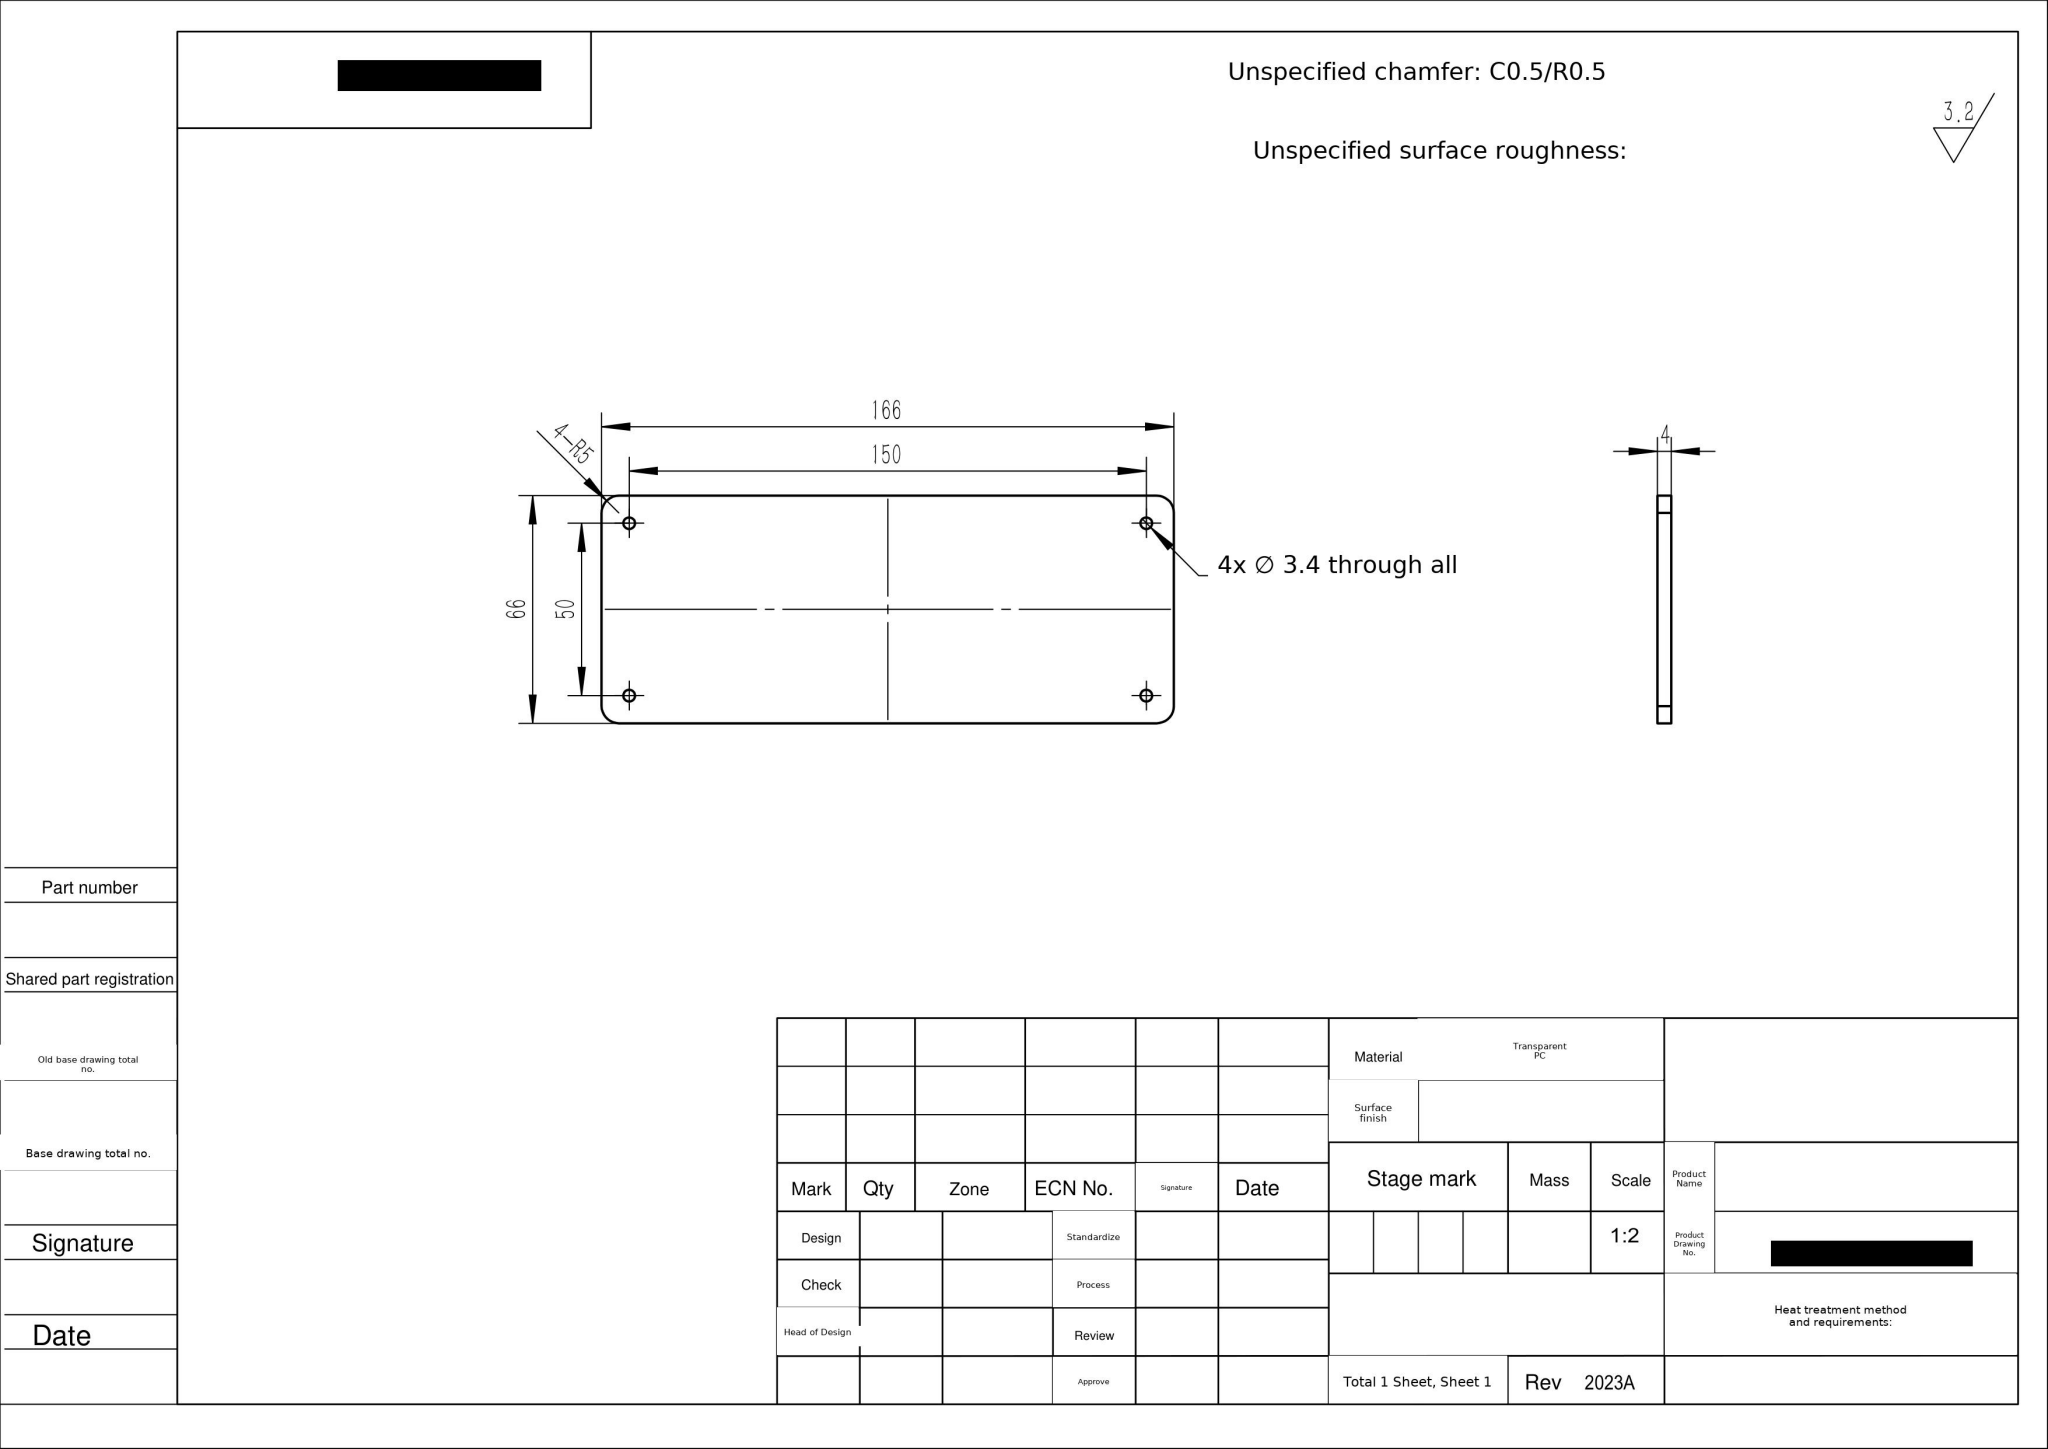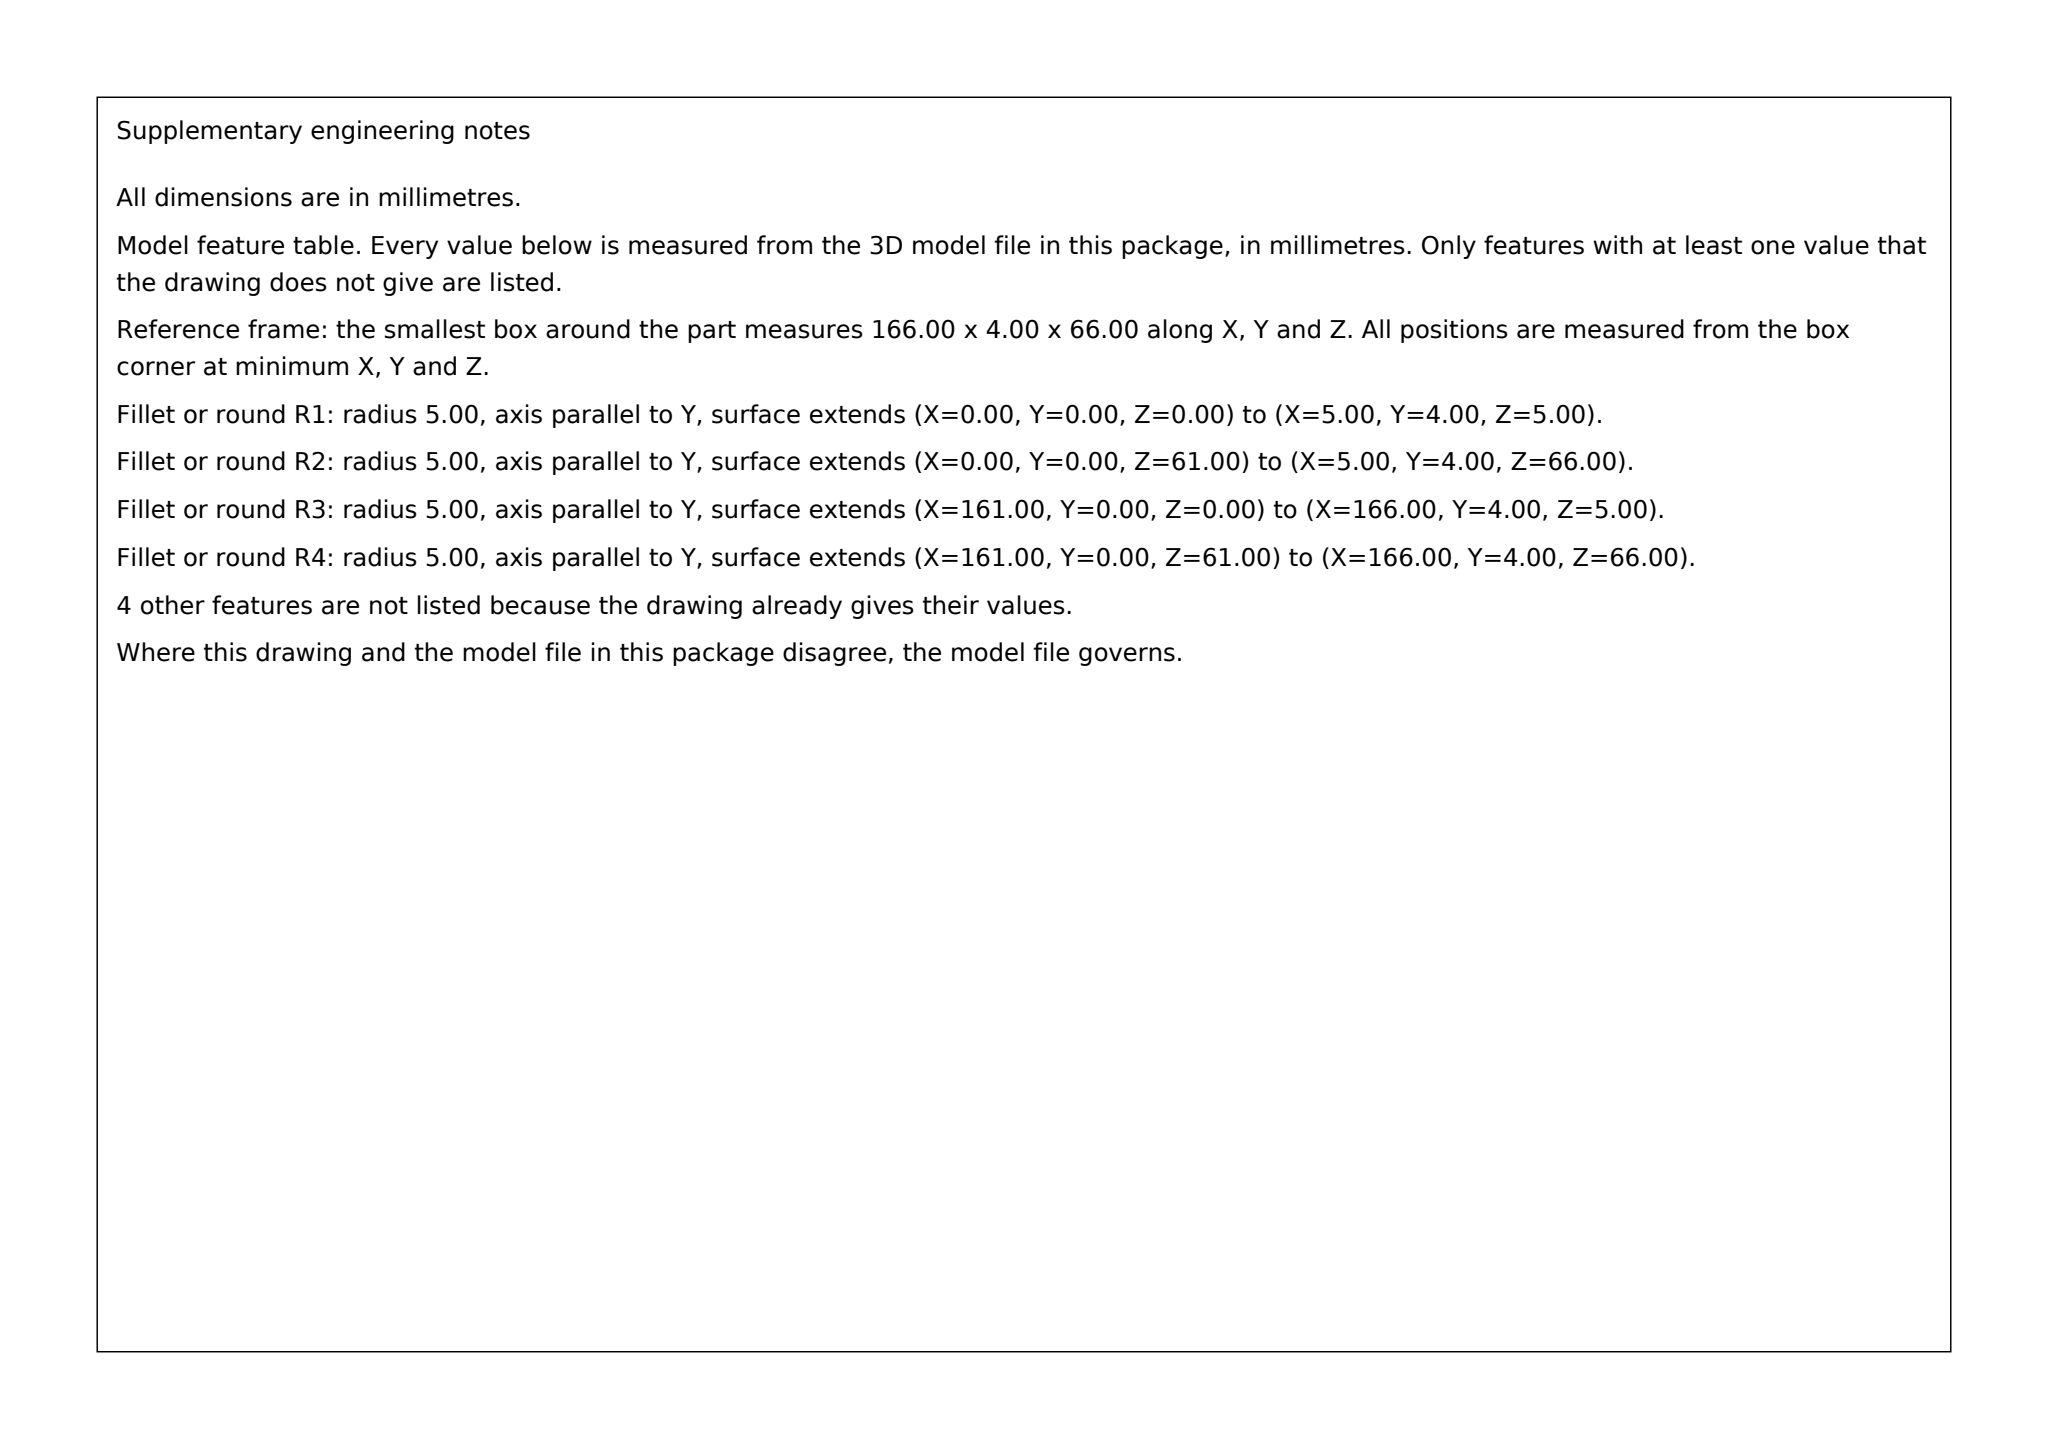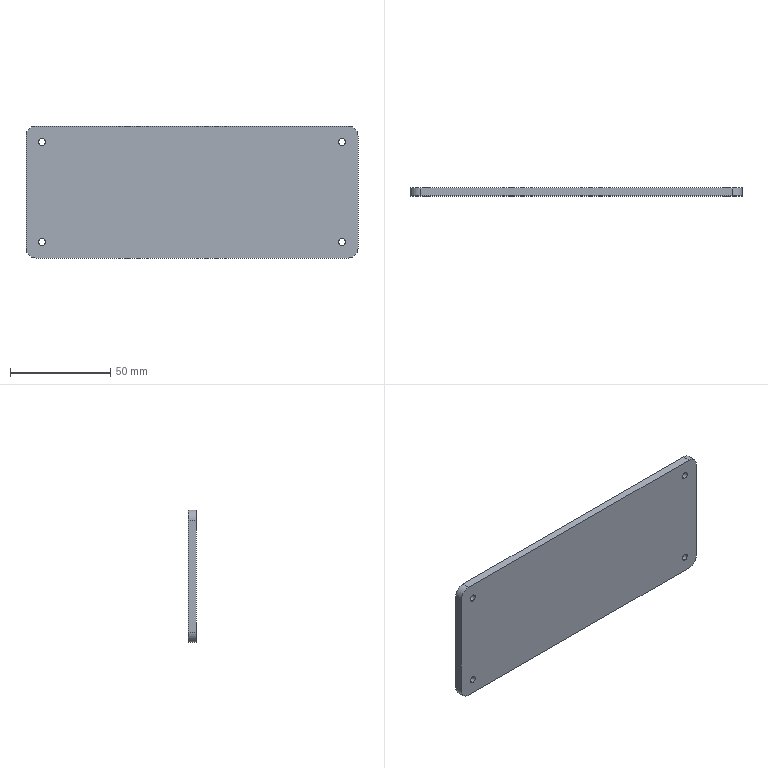Part | SolidWorks | mm | material Transparent PC | 1 solid | 18 faces | box 166 x 4 x 66 mm | volume 43593 mm3 | cylinder 12 | plane 6 | commonest cylinder face diameters 3.4 x8 10 x4
build123d program:
from build123d import *

# Parameters (mm, degrees)
SKETCH1_W            = 166
SKETCH1_H            = 66
BOSS_EXTRUDE1_DEPTH  = 4
M3_CLEARANCE_HOLE1_D = 3.4
FILLET1_R            = 5


with BuildPart() as part:
    # Sketch1 → Boss-Extrude1 (new body)
    with BuildSketch(Plane(origin=(0, 0, 0), x_dir=(1, 0, 0), z_dir=(0, 1, 0))):
        Rectangle(SKETCH1_W, SKETCH1_H)
    extrude(amount=BOSS_EXTRUDE1_DEPTH)

    # M3 Clearance Hole1 (through all)
    with Locations(Plane(origin=(0, 4, 0), x_dir=(-1, 0, 0), z_dir=(0, 1, 0))):
        with Locations((75, -25), (75, 25), (-75, 25), (-75, -25)):
            Hole(M3_CLEARANCE_HOLE1_D / 2)

    # Fillet1
    fillet1_edges = [part.edges().sort_by_distance(p)[0] for p in [
        (83, 2, 33),
        (-83, 2, 33),
        (-83, 2, -33),
        (83, 2, -33),
    ]]
    fillet(fillet1_edges, radius=FILLET1_R)


solid = part.part
STEP:
#1=CARTESIAN_POINT('',(-75.,0.,-26.7));
#2=VERTEX_POINT('',#1);
#3=CARTESIAN_POINT('',(-75.,0.,-23.3));
#4=VERTEX_POINT('',#3);
#5=CARTESIAN_POINT('',(-75.,0.,-25.));
#6=DIRECTION('',(0.,1.,0.));
#7=DIRECTION('',(0.,0.,1.));
#8=AXIS2_PLACEMENT_3D('',#5,#6,#7);
#9=CIRCLE('',#8,1.7);
#10=EDGE_CURVE('',#2,#4,#9,.T.);
#11=ORIENTED_EDGE('',*,*,#10,.F.);
#12=CARTESIAN_POINT('',(-75.,4.,-26.7));
#13=VERTEX_POINT('',#12);
#14=CARTESIAN_POINT('',(-75.,4.,-26.7));
#15=DIRECTION('',(0.,1.,0.));
#16=VECTOR('',#15,1000.);
#17=LINE('',#14,#16);
#18=EDGE_CURVE('',#2,#13,#17,.T.);
#19=ORIENTED_EDGE('',*,*,#18,.T.);
#20=CARTESIAN_POINT('',(-75.,4.,-23.3));
#21=VERTEX_POINT('',#20);
#22=CARTESIAN_POINT('',(-75.,4.,-25.));
#23=DIRECTION('',(0.,1.,0.));
#24=DIRECTION('',(0.,0.,1.));
#25=AXIS2_PLACEMENT_3D('',#22,#23,#24);
#26=CIRCLE('',#25,1.7);
#27=EDGE_CURVE('',#13,#21,#26,.T.);
#28=ORIENTED_EDGE('',*,*,#27,.T.);
#29=CARTESIAN_POINT('',(-75.,4.,-23.3));
#30=DIRECTION('',(0.,1.,0.));
#31=VECTOR('',#30,1000.);
#32=LINE('',#29,#31);
#33=EDGE_CURVE('',#4,#21,#32,.T.);
#34=ORIENTED_EDGE('',*,*,#33,.F.);
#35=EDGE_LOOP('',(#11,#19,#28,#34));
#36=FACE_OUTER_BOUND('',#35,.T.);
#37=CARTESIAN_POINT('',(-75.,4.,-25.));
#38=DIRECTION('',(0.,1.,0.));
#39=DIRECTION('',(0.,0.,1.));
#40=AXIS2_PLACEMENT_3D('',#37,#38,#39);
#41=CYLINDRICAL_SURFACE('',#40,1.7);
#42=ADVANCED_FACE('',(#36),#41,.F.);
#43=CARTESIAN_POINT('',(-75.,0.,23.3));
#44=VERTEX_POINT('',#43);
#45=CARTESIAN_POINT('',(-75.,0.,26.7));
#46=VERTEX_POINT('',#45);
#47=CARTESIAN_POINT('',(-75.,0.,25.));
#48=DIRECTION('',(0.,1.,0.));
#49=DIRECTION('',(0.,0.,1.));
#50=AXIS2_PLACEMENT_3D('',#47,#48,#49);
#51=CIRCLE('',#50,1.7);
#52=EDGE_CURVE('',#44,#46,#51,.T.);
#53=ORIENTED_EDGE('',*,*,#52,.F.);
#54=CARTESIAN_POINT('',(-75.,4.,23.3));
#55=VERTEX_POINT('',#54);
#56=CARTESIAN_POINT('',(-75.,4.,23.3));
#57=DIRECTION('',(0.,1.,0.));
#58=VECTOR('',#57,1000.);
#59=LINE('',#56,#58);
#60=EDGE_CURVE('',#44,#55,#59,.T.);
#61=ORIENTED_EDGE('',*,*,#60,.T.);
#62=CARTESIAN_POINT('',(-75.,4.,26.7));
#63=VERTEX_POINT('',#62);
#64=CARTESIAN_POINT('',(-75.,4.,25.));
#65=DIRECTION('',(0.,1.,0.));
#66=DIRECTION('',(0.,0.,1.));
#67=AXIS2_PLACEMENT_3D('',#64,#65,#66);
#68=CIRCLE('',#67,1.7);
#69=EDGE_CURVE('',#55,#63,#68,.T.);
#70=ORIENTED_EDGE('',*,*,#69,.T.);
#71=CARTESIAN_POINT('',(-75.,4.,26.7));
#72=DIRECTION('',(0.,1.,0.));
#73=VECTOR('',#72,1000.);
#74=LINE('',#71,#73);
#75=EDGE_CURVE('',#46,#63,#74,.T.);
#76=ORIENTED_EDGE('',*,*,#75,.F.);
#77=EDGE_LOOP('',(#53,#61,#70,#76));
#78=FACE_OUTER_BOUND('',#77,.T.);
#79=CARTESIAN_POINT('',(-75.,4.,25.));
#80=DIRECTION('',(0.,1.,0.));
#81=DIRECTION('',(0.,0.,1.));
#82=AXIS2_PLACEMENT_3D('',#79,#80,#81);
#83=CYLINDRICAL_SURFACE('',#82,1.7);
#84=ADVANCED_FACE('',(#78),#83,.F.);
#85=CARTESIAN_POINT('',(75.,0.,23.3));
#86=VERTEX_POINT('',#85);
#87=CARTESIAN_POINT('',(75.,0.,26.7));
#88=VERTEX_POINT('',#87);
#89=CARTESIAN_POINT('',(75.,0.,25.));
#90=DIRECTION('',(0.,1.,0.));
#91=DIRECTION('',(0.,0.,1.));
#92=AXIS2_PLACEMENT_3D('',#89,#90,#91);
#93=CIRCLE('',#92,1.7);
#94=EDGE_CURVE('',#86,#88,#93,.T.);
#95=ORIENTED_EDGE('',*,*,#94,.F.);
#96=CARTESIAN_POINT('',(75.,4.,23.3));
#97=VERTEX_POINT('',#96);
#98=CARTESIAN_POINT('',(75.,4.,23.3));
#99=DIRECTION('',(0.,1.,0.));
#100=VECTOR('',#99,1000.);
#101=LINE('',#98,#100);
#102=EDGE_CURVE('',#86,#97,#101,.T.);
#103=ORIENTED_EDGE('',*,*,#102,.T.);
#104=CARTESIAN_POINT('',(75.,4.,26.7));
#105=VERTEX_POINT('',#104);
#106=CARTESIAN_POINT('',(75.,4.,25.));
#107=DIRECTION('',(0.,1.,0.));
#108=DIRECTION('',(0.,0.,1.));
#109=AXIS2_PLACEMENT_3D('',#106,#107,#108);
#110=CIRCLE('',#109,1.7);
#111=EDGE_CURVE('',#97,#105,#110,.T.);
#112=ORIENTED_EDGE('',*,*,#111,.T.);
#113=CARTESIAN_POINT('',(75.,4.,26.7));
#114=DIRECTION('',(0.,1.,0.));
#115=VECTOR('',#114,1000.);
#116=LINE('',#113,#115);
#117=EDGE_CURVE('',#88,#105,#116,.T.);
#118=ORIENTED_EDGE('',*,*,#117,.F.);
#119=EDGE_LOOP('',(#95,#103,#112,#118));
#120=FACE_OUTER_BOUND('',#119,.T.);
#121=CARTESIAN_POINT('',(75.,4.,25.));
#122=DIRECTION('',(0.,1.,0.));
#123=DIRECTION('',(0.,0.,1.));
#124=AXIS2_PLACEMENT_3D('',#121,#122,#123);
#125=CYLINDRICAL_SURFACE('',#124,1.7);
#126=ADVANCED_FACE('',(#120),#125,.F.);
#127=CARTESIAN_POINT('',(75.,0.,-26.7));
#128=VERTEX_POINT('',#127);
#129=CARTESIAN_POINT('',(75.,0.,-23.3));
#130=VERTEX_POINT('',#129);
#131=CARTESIAN_POINT('',(75.,0.,-25.));
#132=DIRECTION('',(0.,1.,0.));
#133=DIRECTION('',(0.,0.,1.));
#134=AXIS2_PLACEMENT_3D('',#131,#132,#133);
#135=CIRCLE('',#134,1.7);
#136=EDGE_CURVE('',#128,#130,#135,.T.);
#137=ORIENTED_EDGE('',*,*,#136,.F.);
#138=CARTESIAN_POINT('',(75.,4.,-26.7));
#139=VERTEX_POINT('',#138);
#140=CARTESIAN_POINT('',(75.,4.,-26.7));
#141=DIRECTION('',(0.,1.,0.));
#142=VECTOR('',#141,1000.);
#143=LINE('',#140,#142);
#144=EDGE_CURVE('',#128,#139,#143,.T.);
#145=ORIENTED_EDGE('',*,*,#144,.T.);
#146=CARTESIAN_POINT('',(75.,4.,-23.3));
#147=VERTEX_POINT('',#146);
#148=CARTESIAN_POINT('',(75.,4.,-25.));
#149=DIRECTION('',(0.,1.,0.));
#150=DIRECTION('',(0.,0.,1.));
#151=AXIS2_PLACEMENT_3D('',#148,#149,#150);
#152=CIRCLE('',#151,1.7);
#153=EDGE_CURVE('',#139,#147,#152,.T.);
#154=ORIENTED_EDGE('',*,*,#153,.T.);
#155=CARTESIAN_POINT('',(75.,4.,-23.3));
#156=DIRECTION('',(0.,1.,0.));
#157=VECTOR('',#156,1000.);
#158=LINE('',#155,#157);
#159=EDGE_CURVE('',#130,#147,#158,.T.);
#160=ORIENTED_EDGE('',*,*,#159,.F.);
#161=EDGE_LOOP('',(#137,#145,#154,#160));
#162=FACE_OUTER_BOUND('',#161,.T.);
#163=CARTESIAN_POINT('',(75.,4.,-25.));
#164=DIRECTION('',(0.,1.,0.));
#165=DIRECTION('',(0.,0.,1.));
#166=AXIS2_PLACEMENT_3D('',#163,#164,#165);
#167=CYLINDRICAL_SURFACE('',#166,1.7);
#168=ADVANCED_FACE('',(#162),#167,.F.);
#169=CARTESIAN_POINT('',(83.,4.,28.));
#170=VERTEX_POINT('',#169);
#171=CARTESIAN_POINT('',(83.,4.,-28.));
#172=VERTEX_POINT('',#171);
#173=CARTESIAN_POINT('',(83.,4.,33.));
#174=DIRECTION('',(0.,0.,-1.));
#175=VECTOR('',#174,1000.);
#176=LINE('',#173,#175);
#177=EDGE_CURVE('',#170,#172,#176,.T.);
#178=ORIENTED_EDGE('',*,*,#177,.F.);
#179=CARTESIAN_POINT('',(83.,0.,28.));
#180=VERTEX_POINT('',#179);
#181=CARTESIAN_POINT('',(83.,4.,28.));
#182=DIRECTION('',(0.,-1.,0.));
#183=VECTOR('',#182,1000.);
#184=LINE('',#181,#183);
#185=EDGE_CURVE('',#170,#180,#184,.T.);
#186=ORIENTED_EDGE('',*,*,#185,.T.);
#187=CARTESIAN_POINT('',(83.,0.,-28.));
#188=VERTEX_POINT('',#187);
#189=CARTESIAN_POINT('',(83.,0.,33.));
#190=DIRECTION('',(0.,0.,-1.));
#191=VECTOR('',#190,1000.);
#192=LINE('',#189,#191);
#193=EDGE_CURVE('',#180,#188,#192,.T.);
#194=ORIENTED_EDGE('',*,*,#193,.T.);
#195=CARTESIAN_POINT('',(83.,4.,-28.));
#196=DIRECTION('',(0.,1.,0.));
#197=VECTOR('',#196,1000.);
#198=LINE('',#195,#197);
#199=EDGE_CURVE('',#188,#172,#198,.T.);
#200=ORIENTED_EDGE('',*,*,#199,.T.);
#201=EDGE_LOOP('',(#178,#186,#194,#200));
#202=FACE_OUTER_BOUND('',#201,.T.);
#203=CARTESIAN_POINT('',(83.,4.,33.));
#204=DIRECTION('',(-1.,0.,0.));
#205=DIRECTION('',(0.,0.,1.));
#206=AXIS2_PLACEMENT_3D('',#203,#204,#205);
#207=PLANE('',#206);
#208=ADVANCED_FACE('',(#202),#207,.F.);
#209=CARTESIAN_POINT('',(78.,4.,-33.));
#210=VERTEX_POINT('',#209);
#211=CARTESIAN_POINT('',(-78.,4.,-33.));
#212=VERTEX_POINT('',#211);
#213=CARTESIAN_POINT('',(-83.,4.,-33.));
#214=DIRECTION('',(-1.,0.,0.));
#215=VECTOR('',#214,1000.);
#216=LINE('',#213,#215);
#217=EDGE_CURVE('',#210,#212,#216,.T.);
#218=ORIENTED_EDGE('',*,*,#217,.F.);
#219=CARTESIAN_POINT('',(78.,0.,-33.));
#220=VERTEX_POINT('',#219);
#221=CARTESIAN_POINT('',(78.,4.,-33.));
#222=DIRECTION('',(0.,-1.,0.));
#223=VECTOR('',#222,1000.);
#224=LINE('',#221,#223);
#225=EDGE_CURVE('',#210,#220,#224,.T.);
#226=ORIENTED_EDGE('',*,*,#225,.T.);
#227=CARTESIAN_POINT('',(-78.,0.,-33.));
#228=VERTEX_POINT('',#227);
#229=CARTESIAN_POINT('',(-83.,0.,-33.));
#230=DIRECTION('',(-1.,0.,0.));
#231=VECTOR('',#230,1000.);
#232=LINE('',#229,#231);
#233=EDGE_CURVE('',#220,#228,#232,.T.);
#234=ORIENTED_EDGE('',*,*,#233,.T.);
#235=CARTESIAN_POINT('',(-78.,4.,-33.));
#236=DIRECTION('',(0.,1.,0.));
#237=VECTOR('',#236,1000.);
#238=LINE('',#235,#237);
#239=EDGE_CURVE('',#228,#212,#238,.T.);
#240=ORIENTED_EDGE('',*,*,#239,.T.);
#241=EDGE_LOOP('',(#218,#226,#234,#240));
#242=FACE_OUTER_BOUND('',#241,.T.);
#243=CARTESIAN_POINT('',(-83.,4.,-33.));
#244=DIRECTION('',(0.,0.,1.));
#245=DIRECTION('',(1.,0.,0.));
#246=AXIS2_PLACEMENT_3D('',#243,#244,#245);
#247=PLANE('',#246);
#248=ADVANCED_FACE('',(#242),#247,.F.);
#249=CARTESIAN_POINT('',(-83.,4.,-28.));
#250=VERTEX_POINT('',#249);
#251=CARTESIAN_POINT('',(-83.,4.,28.));
#252=VERTEX_POINT('',#251);
#253=CARTESIAN_POINT('',(-83.,4.,33.));
#254=DIRECTION('',(0.,0.,1.));
#255=VECTOR('',#254,1000.);
#256=LINE('',#253,#255);
#257=EDGE_CURVE('',#250,#252,#256,.T.);
#258=ORIENTED_EDGE('',*,*,#257,.F.);
#259=CARTESIAN_POINT('',(-83.,0.,-28.));
#260=VERTEX_POINT('',#259);
#261=CARTESIAN_POINT('',(-83.,4.,-28.));
#262=DIRECTION('',(0.,-1.,0.));
#263=VECTOR('',#262,1000.);
#264=LINE('',#261,#263);
#265=EDGE_CURVE('',#250,#260,#264,.T.);
#266=ORIENTED_EDGE('',*,*,#265,.T.);
#267=CARTESIAN_POINT('',(-83.,0.,28.));
#268=VERTEX_POINT('',#267);
#269=CARTESIAN_POINT('',(-83.,0.,33.));
#270=DIRECTION('',(0.,0.,1.));
#271=VECTOR('',#270,1000.);
#272=LINE('',#269,#271);
#273=EDGE_CURVE('',#260,#268,#272,.T.);
#274=ORIENTED_EDGE('',*,*,#273,.T.);
#275=CARTESIAN_POINT('',(-83.,4.,28.));
#276=DIRECTION('',(0.,1.,0.));
#277=VECTOR('',#276,1000.);
#278=LINE('',#275,#277);
#279=EDGE_CURVE('',#268,#252,#278,.T.);
#280=ORIENTED_EDGE('',*,*,#279,.T.);
#281=EDGE_LOOP('',(#258,#266,#274,#280));
#282=FACE_OUTER_BOUND('',#281,.T.);
#283=CARTESIAN_POINT('',(-83.,4.,33.));
#284=DIRECTION('',(1.,0.,0.));
#285=DIRECTION('',(0.,0.,-1.));
#286=AXIS2_PLACEMENT_3D('',#283,#284,#285);
#287=PLANE('',#286);
#288=ADVANCED_FACE('',(#282),#287,.F.);
#289=CARTESIAN_POINT('',(-78.,0.,33.));
#290=VERTEX_POINT('',#289);
#291=CARTESIAN_POINT('',(78.,0.,33.));
#292=VERTEX_POINT('',#291);
#293=CARTESIAN_POINT('',(-83.,0.,33.));
#294=DIRECTION('',(1.,0.,0.));
#295=VECTOR('',#294,1000.);
#296=LINE('',#293,#295);
#297=EDGE_CURVE('',#290,#292,#296,.T.);
#298=ORIENTED_EDGE('',*,*,#297,.T.);
#299=CARTESIAN_POINT('',(78.,4.,33.));
#300=VERTEX_POINT('',#299);
#301=CARTESIAN_POINT('',(78.,4.,33.));
#302=DIRECTION('',(0.,1.,0.));
#303=VECTOR('',#302,1000.);
#304=LINE('',#301,#303);
#305=EDGE_CURVE('',#292,#300,#304,.T.);
#306=ORIENTED_EDGE('',*,*,#305,.T.);
#307=CARTESIAN_POINT('',(-78.,4.,33.));
#308=VERTEX_POINT('',#307);
#309=CARTESIAN_POINT('',(-83.,4.,33.));
#310=DIRECTION('',(1.,0.,0.));
#311=VECTOR('',#310,1000.);
#312=LINE('',#309,#311);
#313=EDGE_CURVE('',#308,#300,#312,.T.);
#314=ORIENTED_EDGE('',*,*,#313,.F.);
#315=CARTESIAN_POINT('',(-78.,4.,33.));
#316=DIRECTION('',(0.,-1.,0.));
#317=VECTOR('',#316,1000.);
#318=LINE('',#315,#317);
#319=EDGE_CURVE('',#308,#290,#318,.T.);
#320=ORIENTED_EDGE('',*,*,#319,.T.);
#321=EDGE_LOOP('',(#298,#306,#314,#320));
#322=FACE_OUTER_BOUND('',#321,.T.);
#323=CARTESIAN_POINT('',(-83.,4.,33.));
#324=DIRECTION('',(0.,0.,-1.));
#325=DIRECTION('',(-1.,0.,0.));
#326=AXIS2_PLACEMENT_3D('',#323,#324,#325);
#327=PLANE('',#326);
#328=ADVANCED_FACE('',(#322),#327,.F.);
#329=CARTESIAN_POINT('',(-75.,4.,-25.));
#330=DIRECTION('',(0.,1.,0.));
#331=DIRECTION('',(0.,0.,1.));
#332=AXIS2_PLACEMENT_3D('',#329,#330,#331);
#333=CIRCLE('',#332,1.7);
#334=EDGE_CURVE('',#21,#13,#333,.T.);
#335=ORIENTED_EDGE('',*,*,#334,.F.);
#336=ORIENTED_EDGE('',*,*,#27,.F.);
#337=EDGE_LOOP('',(#335,#336));
#338=FACE_BOUND('',#337,.T.);
#339=CARTESIAN_POINT('',(-75.,4.,25.));
#340=DIRECTION('',(0.,1.,0.));
#341=DIRECTION('',(0.,0.,1.));
#342=AXIS2_PLACEMENT_3D('',#339,#340,#341);
#343=CIRCLE('',#342,1.7);
#344=EDGE_CURVE('',#63,#55,#343,.T.);
#345=ORIENTED_EDGE('',*,*,#344,.F.);
#346=ORIENTED_EDGE('',*,*,#69,.F.);
#347=EDGE_LOOP('',(#345,#346));
#348=FACE_BOUND('',#347,.T.);
#349=CARTESIAN_POINT('',(75.,4.,25.));
#350=DIRECTION('',(0.,1.,0.));
#351=DIRECTION('',(0.,0.,1.));
#352=AXIS2_PLACEMENT_3D('',#349,#350,#351);
#353=CIRCLE('',#352,1.7);
#354=EDGE_CURVE('',#105,#97,#353,.T.);
#355=ORIENTED_EDGE('',*,*,#354,.F.);
#356=ORIENTED_EDGE('',*,*,#111,.F.);
#357=EDGE_LOOP('',(#355,#356));
#358=FACE_BOUND('',#357,.T.);
#359=CARTESIAN_POINT('',(75.,4.,-25.));
#360=DIRECTION('',(0.,1.,0.));
#361=DIRECTION('',(0.,0.,1.));
#362=AXIS2_PLACEMENT_3D('',#359,#360,#361);
#363=CIRCLE('',#362,1.7);
#364=EDGE_CURVE('',#147,#139,#363,.T.);
#365=ORIENTED_EDGE('',*,*,#364,.F.);
#366=ORIENTED_EDGE('',*,*,#153,.F.);
#367=EDGE_LOOP('',(#365,#366));
#368=FACE_BOUND('',#367,.T.);
#369=ORIENTED_EDGE('',*,*,#313,.T.);
#370=CARTESIAN_POINT('',(78.,4.,28.));
#371=DIRECTION('',(0.,1.,0.));
#372=DIRECTION('',(0.,0.,-1.));
#373=AXIS2_PLACEMENT_3D('',#370,#371,#372);
#374=CIRCLE('',#373,5.);
#375=EDGE_CURVE('',#300,#170,#374,.T.);
#376=ORIENTED_EDGE('',*,*,#375,.T.);
#377=ORIENTED_EDGE('',*,*,#177,.T.);
#378=CARTESIAN_POINT('',(78.,4.,-28.));
#379=DIRECTION('',(0.,1.,0.));
#380=DIRECTION('',(0.,0.,-1.));
#381=AXIS2_PLACEMENT_3D('',#378,#379,#380);
#382=CIRCLE('',#381,5.);
#383=EDGE_CURVE('',#172,#210,#382,.T.);
#384=ORIENTED_EDGE('',*,*,#383,.T.);
#385=ORIENTED_EDGE('',*,*,#217,.T.);
#386=CARTESIAN_POINT('',(-78.,4.,-28.));
#387=DIRECTION('',(0.,1.,0.));
#388=DIRECTION('',(0.,0.,-1.));
#389=AXIS2_PLACEMENT_3D('',#386,#387,#388);
#390=CIRCLE('',#389,5.);
#391=EDGE_CURVE('',#212,#250,#390,.T.);
#392=ORIENTED_EDGE('',*,*,#391,.T.);
#393=ORIENTED_EDGE('',*,*,#257,.T.);
#394=CARTESIAN_POINT('',(-78.,4.,28.));
#395=DIRECTION('',(0.,1.,0.));
#396=DIRECTION('',(0.,0.,-1.));
#397=AXIS2_PLACEMENT_3D('',#394,#395,#396);
#398=CIRCLE('',#397,5.);
#399=EDGE_CURVE('',#252,#308,#398,.T.);
#400=ORIENTED_EDGE('',*,*,#399,.T.);
#401=EDGE_LOOP('',(#369,#376,#377,#384,#385,#392,#393,#400));
#402=FACE_OUTER_BOUND('',#401,.T.);
#403=CARTESIAN_POINT('',(0.,4.,0.));
#404=DIRECTION('',(0.,-1.,0.));
#405=DIRECTION('',(0.,0.,-1.));
#406=AXIS2_PLACEMENT_3D('',#403,#404,#405);
#407=PLANE('',#406);
#408=ADVANCED_FACE('',(#338,#348,#358,#368,#402),#407,.F.);
#409=CARTESIAN_POINT('',(-75.,0.,-25.));
#410=DIRECTION('',(0.,1.,0.));
#411=DIRECTION('',(0.,0.,1.));
#412=AXIS2_PLACEMENT_3D('',#409,#410,#411);
#413=CIRCLE('',#412,1.7);
#414=EDGE_CURVE('',#4,#2,#413,.T.);
#415=ORIENTED_EDGE('',*,*,#414,.T.);
#416=ORIENTED_EDGE('',*,*,#10,.T.);
#417=EDGE_LOOP('',(#415,#416));
#418=FACE_BOUND('',#417,.T.);
#419=CARTESIAN_POINT('',(-75.,0.,25.));
#420=DIRECTION('',(0.,1.,0.));
#421=DIRECTION('',(0.,0.,1.));
#422=AXIS2_PLACEMENT_3D('',#419,#420,#421);
#423=CIRCLE('',#422,1.7);
#424=EDGE_CURVE('',#46,#44,#423,.T.);
#425=ORIENTED_EDGE('',*,*,#424,.T.);
#426=ORIENTED_EDGE('',*,*,#52,.T.);
#427=EDGE_LOOP('',(#425,#426));
#428=FACE_BOUND('',#427,.T.);
#429=CARTESIAN_POINT('',(75.,0.,25.));
#430=DIRECTION('',(0.,1.,0.));
#431=DIRECTION('',(0.,0.,1.));
#432=AXIS2_PLACEMENT_3D('',#429,#430,#431);
#433=CIRCLE('',#432,1.7);
#434=EDGE_CURVE('',#88,#86,#433,.T.);
#435=ORIENTED_EDGE('',*,*,#434,.T.);
#436=ORIENTED_EDGE('',*,*,#94,.T.);
#437=EDGE_LOOP('',(#435,#436));
#438=FACE_BOUND('',#437,.T.);
#439=CARTESIAN_POINT('',(75.,0.,-25.));
#440=DIRECTION('',(0.,1.,0.));
#441=DIRECTION('',(0.,0.,1.));
#442=AXIS2_PLACEMENT_3D('',#439,#440,#441);
#443=CIRCLE('',#442,1.7);
#444=EDGE_CURVE('',#130,#128,#443,.T.);
#445=ORIENTED_EDGE('',*,*,#444,.T.);
#446=ORIENTED_EDGE('',*,*,#136,.T.);
#447=EDGE_LOOP('',(#445,#446));
#448=FACE_BOUND('',#447,.T.);
#449=ORIENTED_EDGE('',*,*,#193,.F.);
#450=CARTESIAN_POINT('',(78.,0.,28.));
#451=DIRECTION('',(0.,-1.,0.));
#452=DIRECTION('',(0.,0.,-1.));
#453=AXIS2_PLACEMENT_3D('',#450,#451,#452);
#454=CIRCLE('',#453,5.);
#455=EDGE_CURVE('',#180,#292,#454,.T.);
#456=ORIENTED_EDGE('',*,*,#455,.T.);
#457=ORIENTED_EDGE('',*,*,#297,.F.);
#458=CARTESIAN_POINT('',(-78.,0.,28.));
#459=DIRECTION('',(0.,-1.,0.));
#460=DIRECTION('',(0.,0.,-1.));
#461=AXIS2_PLACEMENT_3D('',#458,#459,#460);
#462=CIRCLE('',#461,5.);
#463=EDGE_CURVE('',#290,#268,#462,.T.);
#464=ORIENTED_EDGE('',*,*,#463,.T.);
#465=ORIENTED_EDGE('',*,*,#273,.F.);
#466=CARTESIAN_POINT('',(-78.,0.,-28.));
#467=DIRECTION('',(0.,-1.,0.));
#468=DIRECTION('',(0.,0.,-1.));
#469=AXIS2_PLACEMENT_3D('',#466,#467,#468);
#470=CIRCLE('',#469,5.);
#471=EDGE_CURVE('',#260,#228,#470,.T.);
#472=ORIENTED_EDGE('',*,*,#471,.T.);
#473=ORIENTED_EDGE('',*,*,#233,.F.);
#474=CARTESIAN_POINT('',(78.,0.,-28.));
#475=DIRECTION('',(0.,-1.,0.));
#476=DIRECTION('',(0.,0.,-1.));
#477=AXIS2_PLACEMENT_3D('',#474,#475,#476);
#478=CIRCLE('',#477,5.);
#479=EDGE_CURVE('',#220,#188,#478,.T.);
#480=ORIENTED_EDGE('',*,*,#479,.T.);
#481=EDGE_LOOP('',(#449,#456,#457,#464,#465,#472,#473,#480));
#482=FACE_OUTER_BOUND('',#481,.T.);
#483=CARTESIAN_POINT('',(0.,0.,0.));
#484=DIRECTION('',(0.,-1.,0.));
#485=DIRECTION('',(0.,0.,-1.));
#486=AXIS2_PLACEMENT_3D('',#483,#484,#485);
#487=PLANE('',#486);
#488=ADVANCED_FACE('',(#418,#428,#438,#448,#482),#487,.T.);
#489=ORIENTED_EDGE('',*,*,#144,.F.);
#490=ORIENTED_EDGE('',*,*,#444,.F.);
#491=ORIENTED_EDGE('',*,*,#159,.T.);
#492=ORIENTED_EDGE('',*,*,#364,.T.);
#493=EDGE_LOOP('',(#489,#490,#491,#492));
#494=FACE_OUTER_BOUND('',#493,.T.);
#495=CARTESIAN_POINT('',(75.,4.,-25.));
#496=DIRECTION('',(0.,1.,0.));
#497=DIRECTION('',(0.,0.,1.));
#498=AXIS2_PLACEMENT_3D('',#495,#496,#497);
#499=CYLINDRICAL_SURFACE('',#498,1.7);
#500=ADVANCED_FACE('',(#494),#499,.F.);
#501=ORIENTED_EDGE('',*,*,#102,.F.);
#502=ORIENTED_EDGE('',*,*,#434,.F.);
#503=ORIENTED_EDGE('',*,*,#117,.T.);
#504=ORIENTED_EDGE('',*,*,#354,.T.);
#505=EDGE_LOOP('',(#501,#502,#503,#504));
#506=FACE_OUTER_BOUND('',#505,.T.);
#507=CARTESIAN_POINT('',(75.,4.,25.));
#508=DIRECTION('',(0.,1.,0.));
#509=DIRECTION('',(0.,0.,1.));
#510=AXIS2_PLACEMENT_3D('',#507,#508,#509);
#511=CYLINDRICAL_SURFACE('',#510,1.7);
#512=ADVANCED_FACE('',(#506),#511,.F.);
#513=ORIENTED_EDGE('',*,*,#60,.F.);
#514=ORIENTED_EDGE('',*,*,#424,.F.);
#515=ORIENTED_EDGE('',*,*,#75,.T.);
#516=ORIENTED_EDGE('',*,*,#344,.T.);
#517=EDGE_LOOP('',(#513,#514,#515,#516));
#518=FACE_OUTER_BOUND('',#517,.T.);
#519=CARTESIAN_POINT('',(-75.,4.,25.));
#520=DIRECTION('',(0.,1.,0.));
#521=DIRECTION('',(0.,0.,1.));
#522=AXIS2_PLACEMENT_3D('',#519,#520,#521);
#523=CYLINDRICAL_SURFACE('',#522,1.7);
#524=ADVANCED_FACE('',(#518),#523,.F.);
#525=ORIENTED_EDGE('',*,*,#18,.F.);
#526=ORIENTED_EDGE('',*,*,#414,.F.);
#527=ORIENTED_EDGE('',*,*,#33,.T.);
#528=ORIENTED_EDGE('',*,*,#334,.T.);
#529=EDGE_LOOP('',(#525,#526,#527,#528));
#530=FACE_OUTER_BOUND('',#529,.T.);
#531=CARTESIAN_POINT('',(-75.,4.,-25.));
#532=DIRECTION('',(0.,1.,0.));
#533=DIRECTION('',(0.,0.,1.));
#534=AXIS2_PLACEMENT_3D('',#531,#532,#533);
#535=CYLINDRICAL_SURFACE('',#534,1.7);
#536=ADVANCED_FACE('',(#530),#535,.F.);
#537=ORIENTED_EDGE('',*,*,#375,.F.);
#538=ORIENTED_EDGE('',*,*,#305,.F.);
#539=ORIENTED_EDGE('',*,*,#455,.F.);
#540=ORIENTED_EDGE('',*,*,#185,.F.);
#541=EDGE_LOOP('',(#537,#538,#539,#540));
#542=FACE_OUTER_BOUND('',#541,.T.);
#543=CARTESIAN_POINT('',(78.,4.,28.));
#544=DIRECTION('',(0.,-1.,0.));
#545=DIRECTION('',(0.,0.,-1.));
#546=AXIS2_PLACEMENT_3D('',#543,#544,#545);
#547=CYLINDRICAL_SURFACE('',#546,5.);
#548=ADVANCED_FACE('',(#542),#547,.T.);
#549=ORIENTED_EDGE('',*,*,#383,.F.);
#550=ORIENTED_EDGE('',*,*,#199,.F.);
#551=ORIENTED_EDGE('',*,*,#479,.F.);
#552=ORIENTED_EDGE('',*,*,#225,.F.);
#553=EDGE_LOOP('',(#549,#550,#551,#552));
#554=FACE_OUTER_BOUND('',#553,.T.);
#555=CARTESIAN_POINT('',(78.,4.,-28.));
#556=DIRECTION('',(0.,-1.,0.));
#557=DIRECTION('',(0.,0.,-1.));
#558=AXIS2_PLACEMENT_3D('',#555,#556,#557);
#559=CYLINDRICAL_SURFACE('',#558,5.);
#560=ADVANCED_FACE('',(#554),#559,.T.);
#561=ORIENTED_EDGE('',*,*,#391,.F.);
#562=ORIENTED_EDGE('',*,*,#239,.F.);
#563=ORIENTED_EDGE('',*,*,#471,.F.);
#564=ORIENTED_EDGE('',*,*,#265,.F.);
#565=EDGE_LOOP('',(#561,#562,#563,#564));
#566=FACE_OUTER_BOUND('',#565,.T.);
#567=CARTESIAN_POINT('',(-78.,4.,-28.));
#568=DIRECTION('',(0.,-1.,0.));
#569=DIRECTION('',(0.,0.,-1.));
#570=AXIS2_PLACEMENT_3D('',#567,#568,#569);
#571=CYLINDRICAL_SURFACE('',#570,5.);
#572=ADVANCED_FACE('',(#566),#571,.T.);
#573=ORIENTED_EDGE('',*,*,#399,.F.);
#574=ORIENTED_EDGE('',*,*,#279,.F.);
#575=ORIENTED_EDGE('',*,*,#463,.F.);
#576=ORIENTED_EDGE('',*,*,#319,.F.);
#577=EDGE_LOOP('',(#573,#574,#575,#576));
#578=FACE_OUTER_BOUND('',#577,.T.);
#579=CARTESIAN_POINT('',(-78.,4.,28.));
#580=DIRECTION('',(0.,-1.,0.));
#581=DIRECTION('',(0.,0.,-1.));
#582=AXIS2_PLACEMENT_3D('',#579,#580,#581);
#583=CYLINDRICAL_SURFACE('',#582,5.);
#584=ADVANCED_FACE('',(#578),#583,.T.);
#585=CLOSED_SHELL('',(#42,#84,#126,#168,#208,#248,#288,#328,#408,#488,#500,#512,#524,#536,#548,#560,#572,#584));
#586=MANIFOLD_SOLID_BREP('',#585);
#587=CARTESIAN_POINT('',(0.,0.,0.));
#588=DIRECTION('',(0.,0.,1.));
#589=DIRECTION('',(1.,0.,0.));
#590=AXIS2_PLACEMENT_3D('',#587,#588,#589);
#591=(LENGTH_UNIT()NAMED_UNIT(*)SI_UNIT(.MILLI.,.METRE.));
#592=UNCERTAINTY_MEASURE_WITH_UNIT(LENGTH_MEASURE(0.00001),#591,'','');
#593=(NAMED_UNIT(*)PLANE_ANGLE_UNIT()SI_UNIT($,.RADIAN.));
#594=(NAMED_UNIT(*)SI_UNIT($,.STERADIAN.)SOLID_ANGLE_UNIT());
#595=(GEOMETRIC_REPRESENTATION_CONTEXT(3)GLOBAL_UNCERTAINTY_ASSIGNED_CONTEXT((#592))GLOBAL_UNIT_ASSIGNED_CONTEXT((#591,#593,#594))REPRESENTATION_CONTEXT('',''));
#596=ADVANCED_BREP_SHAPE_REPRESENTATION('',(#586,#590),#595);